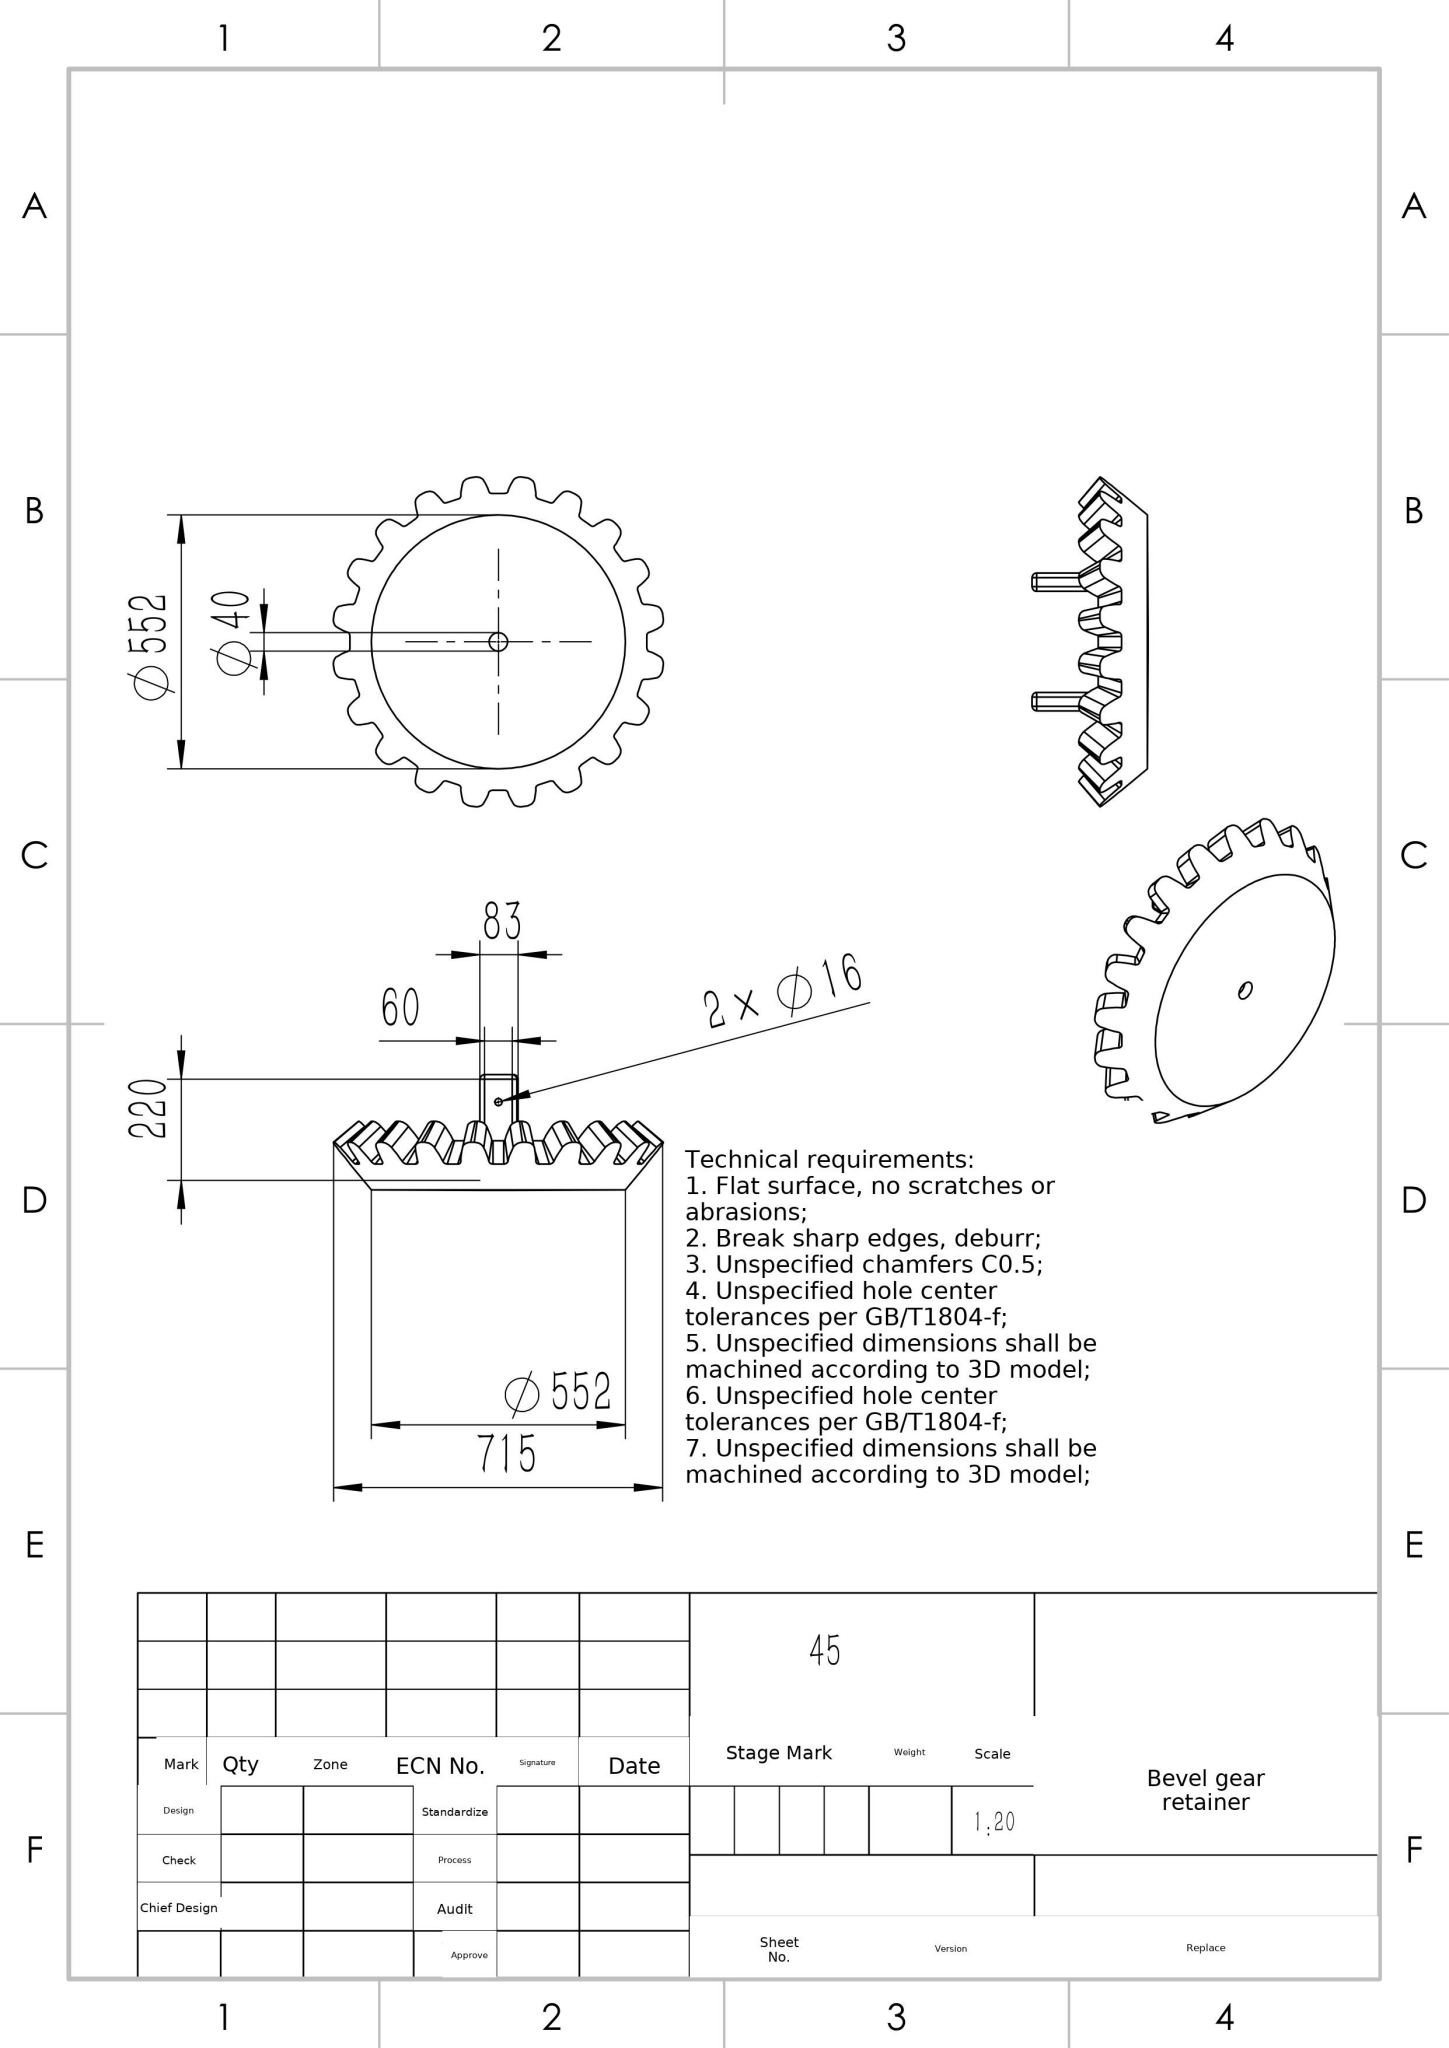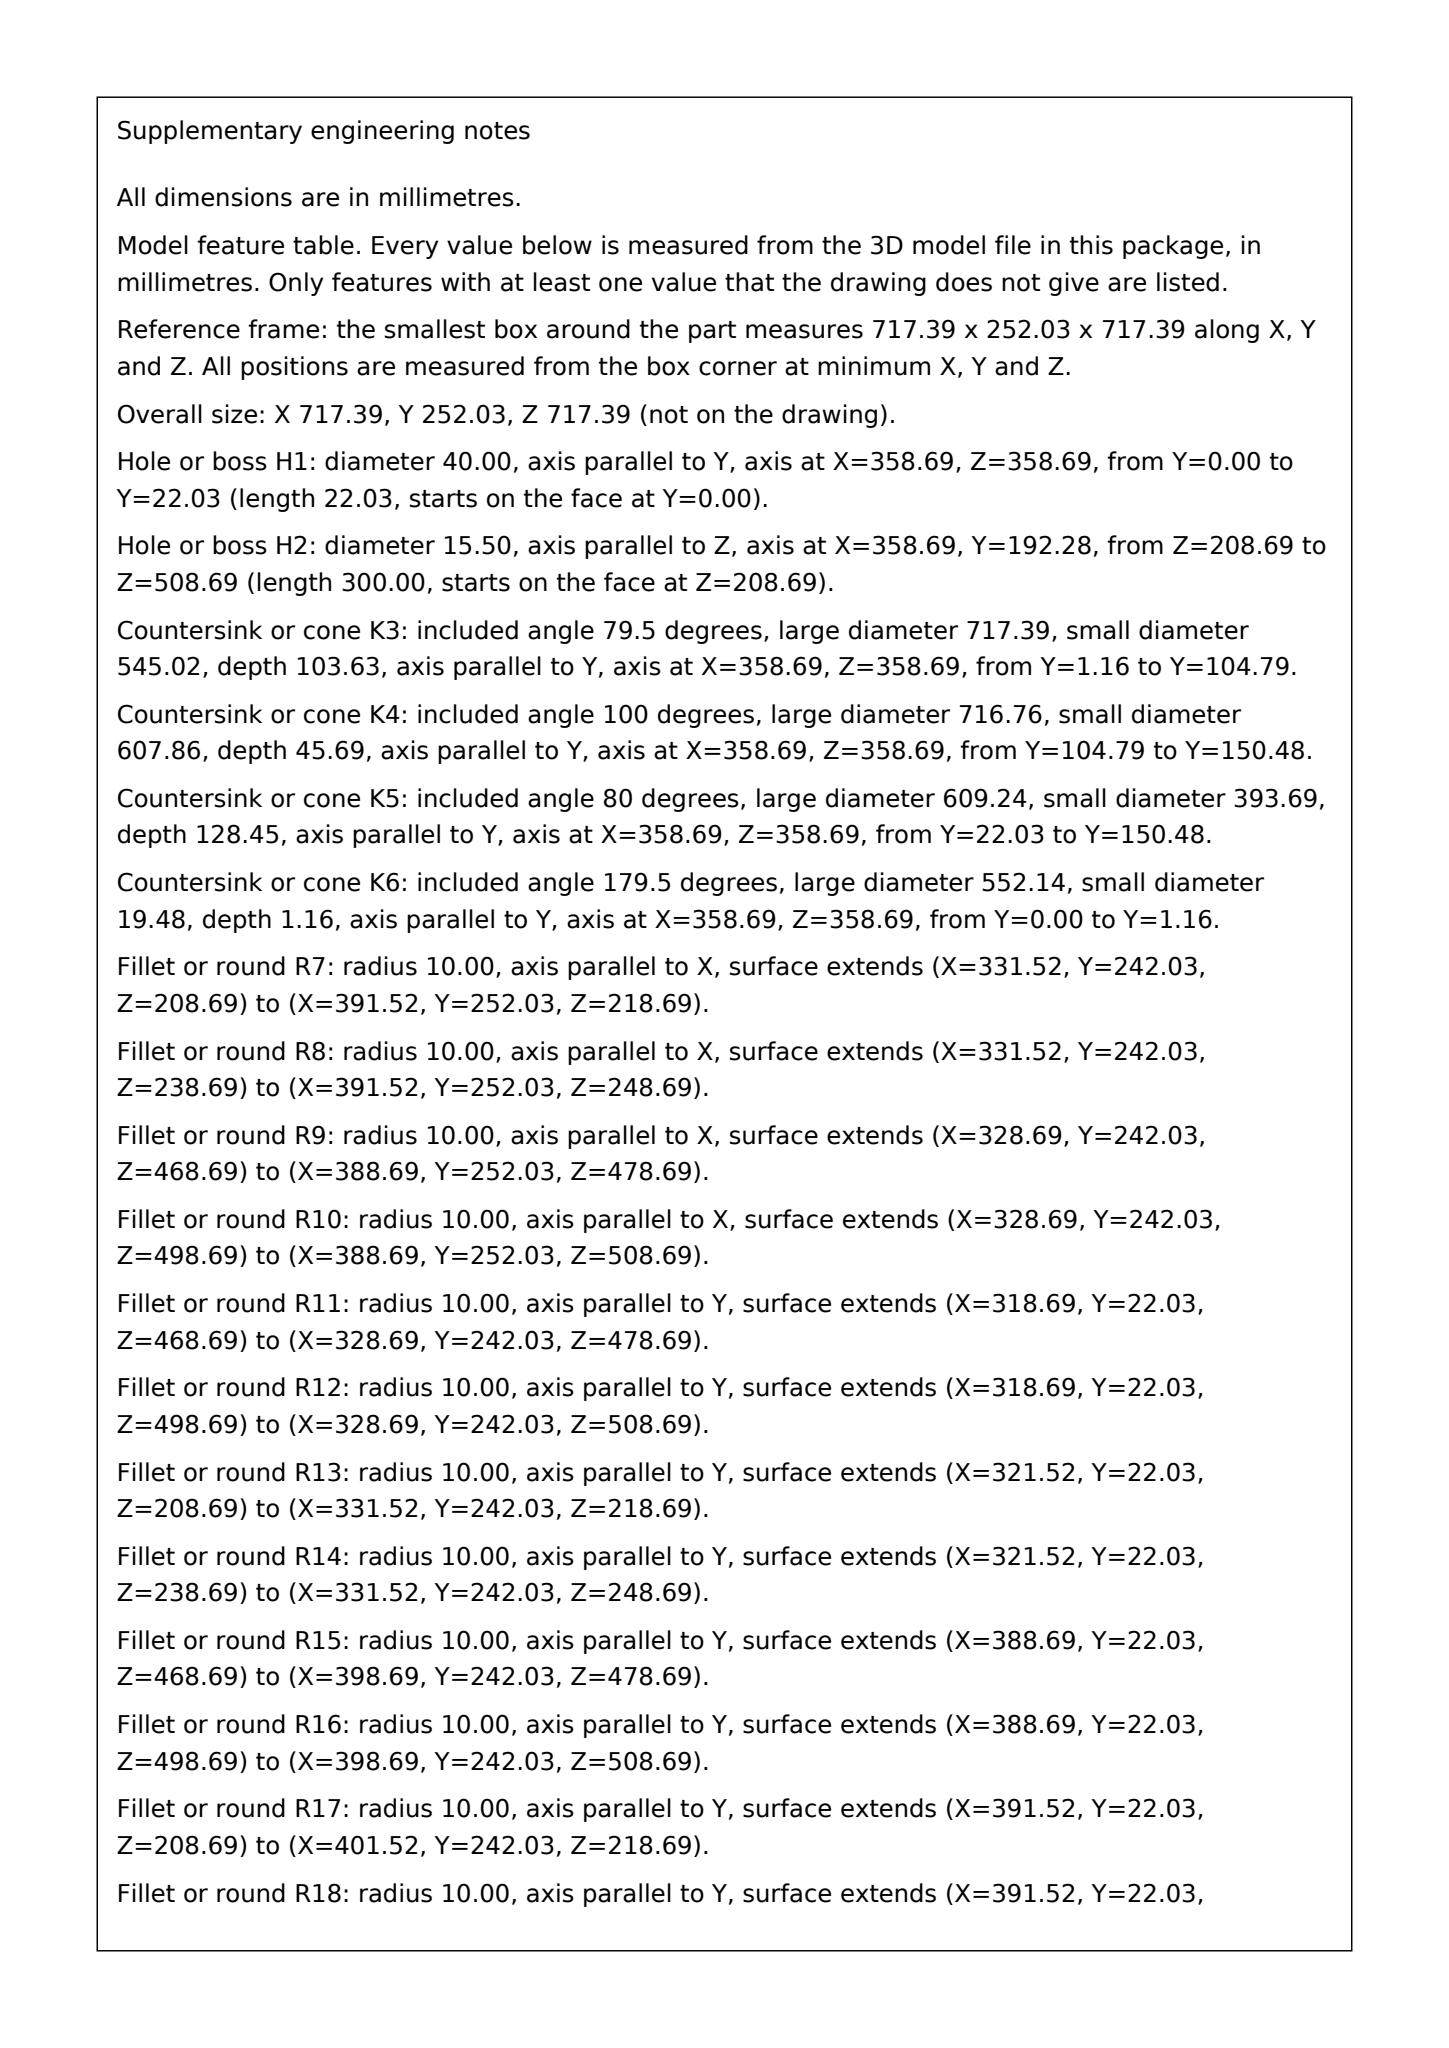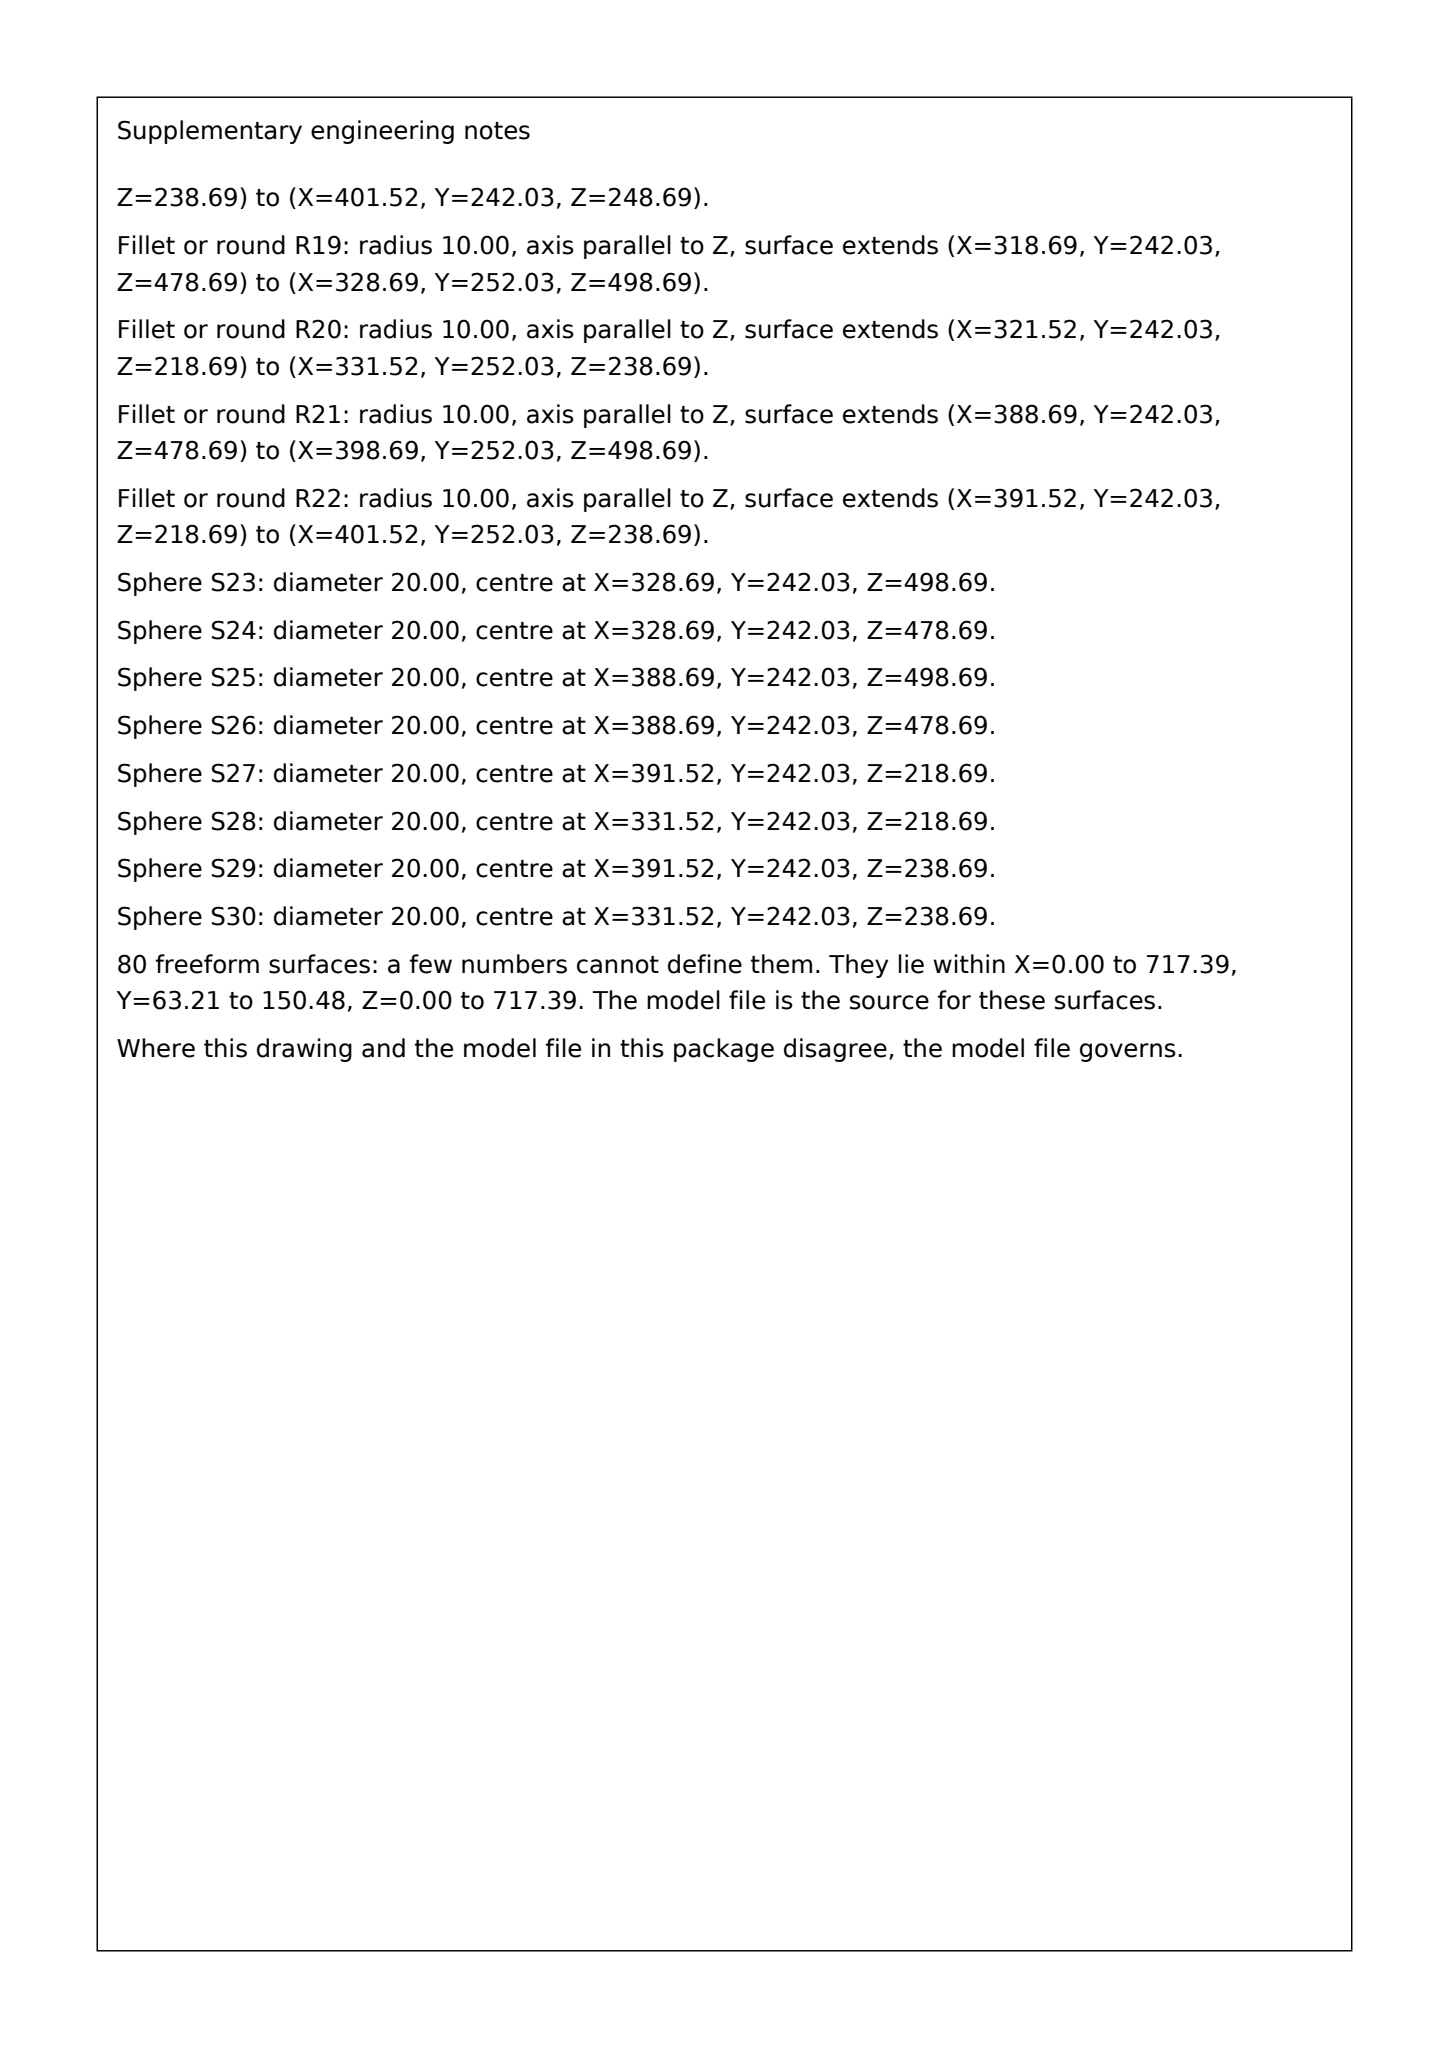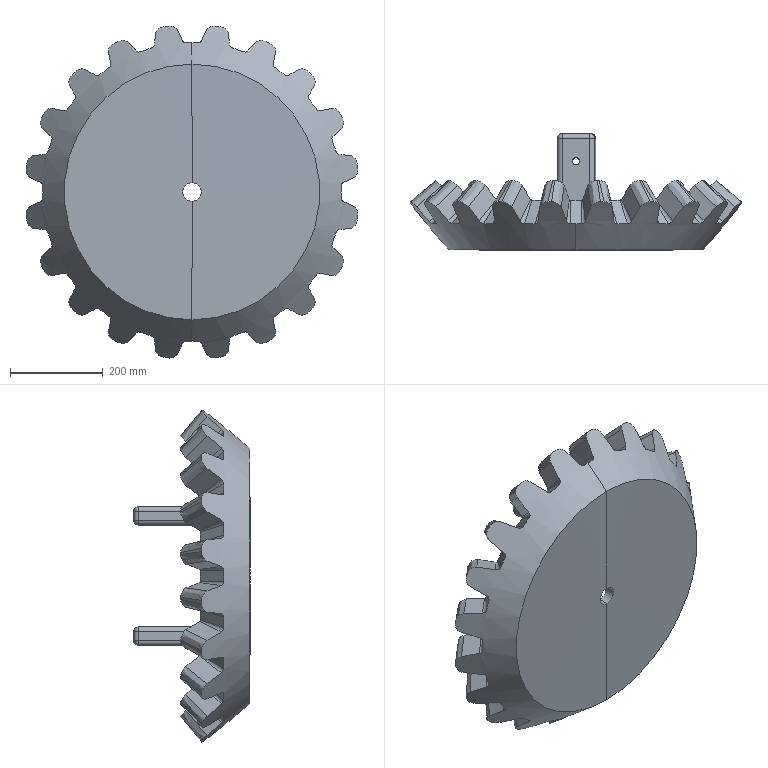Part | SolidWorks | mm | material 45 | 1 solid | 207 faces | box 717.39 x 252.03 x 717.39 mm | volume 20400351 mm3 | spline 80 | cone 66 | plane 31 | cylinder 22 | sphere 8 | commonest cylinder face diameters 20 x16 15.5 x4 40 x2